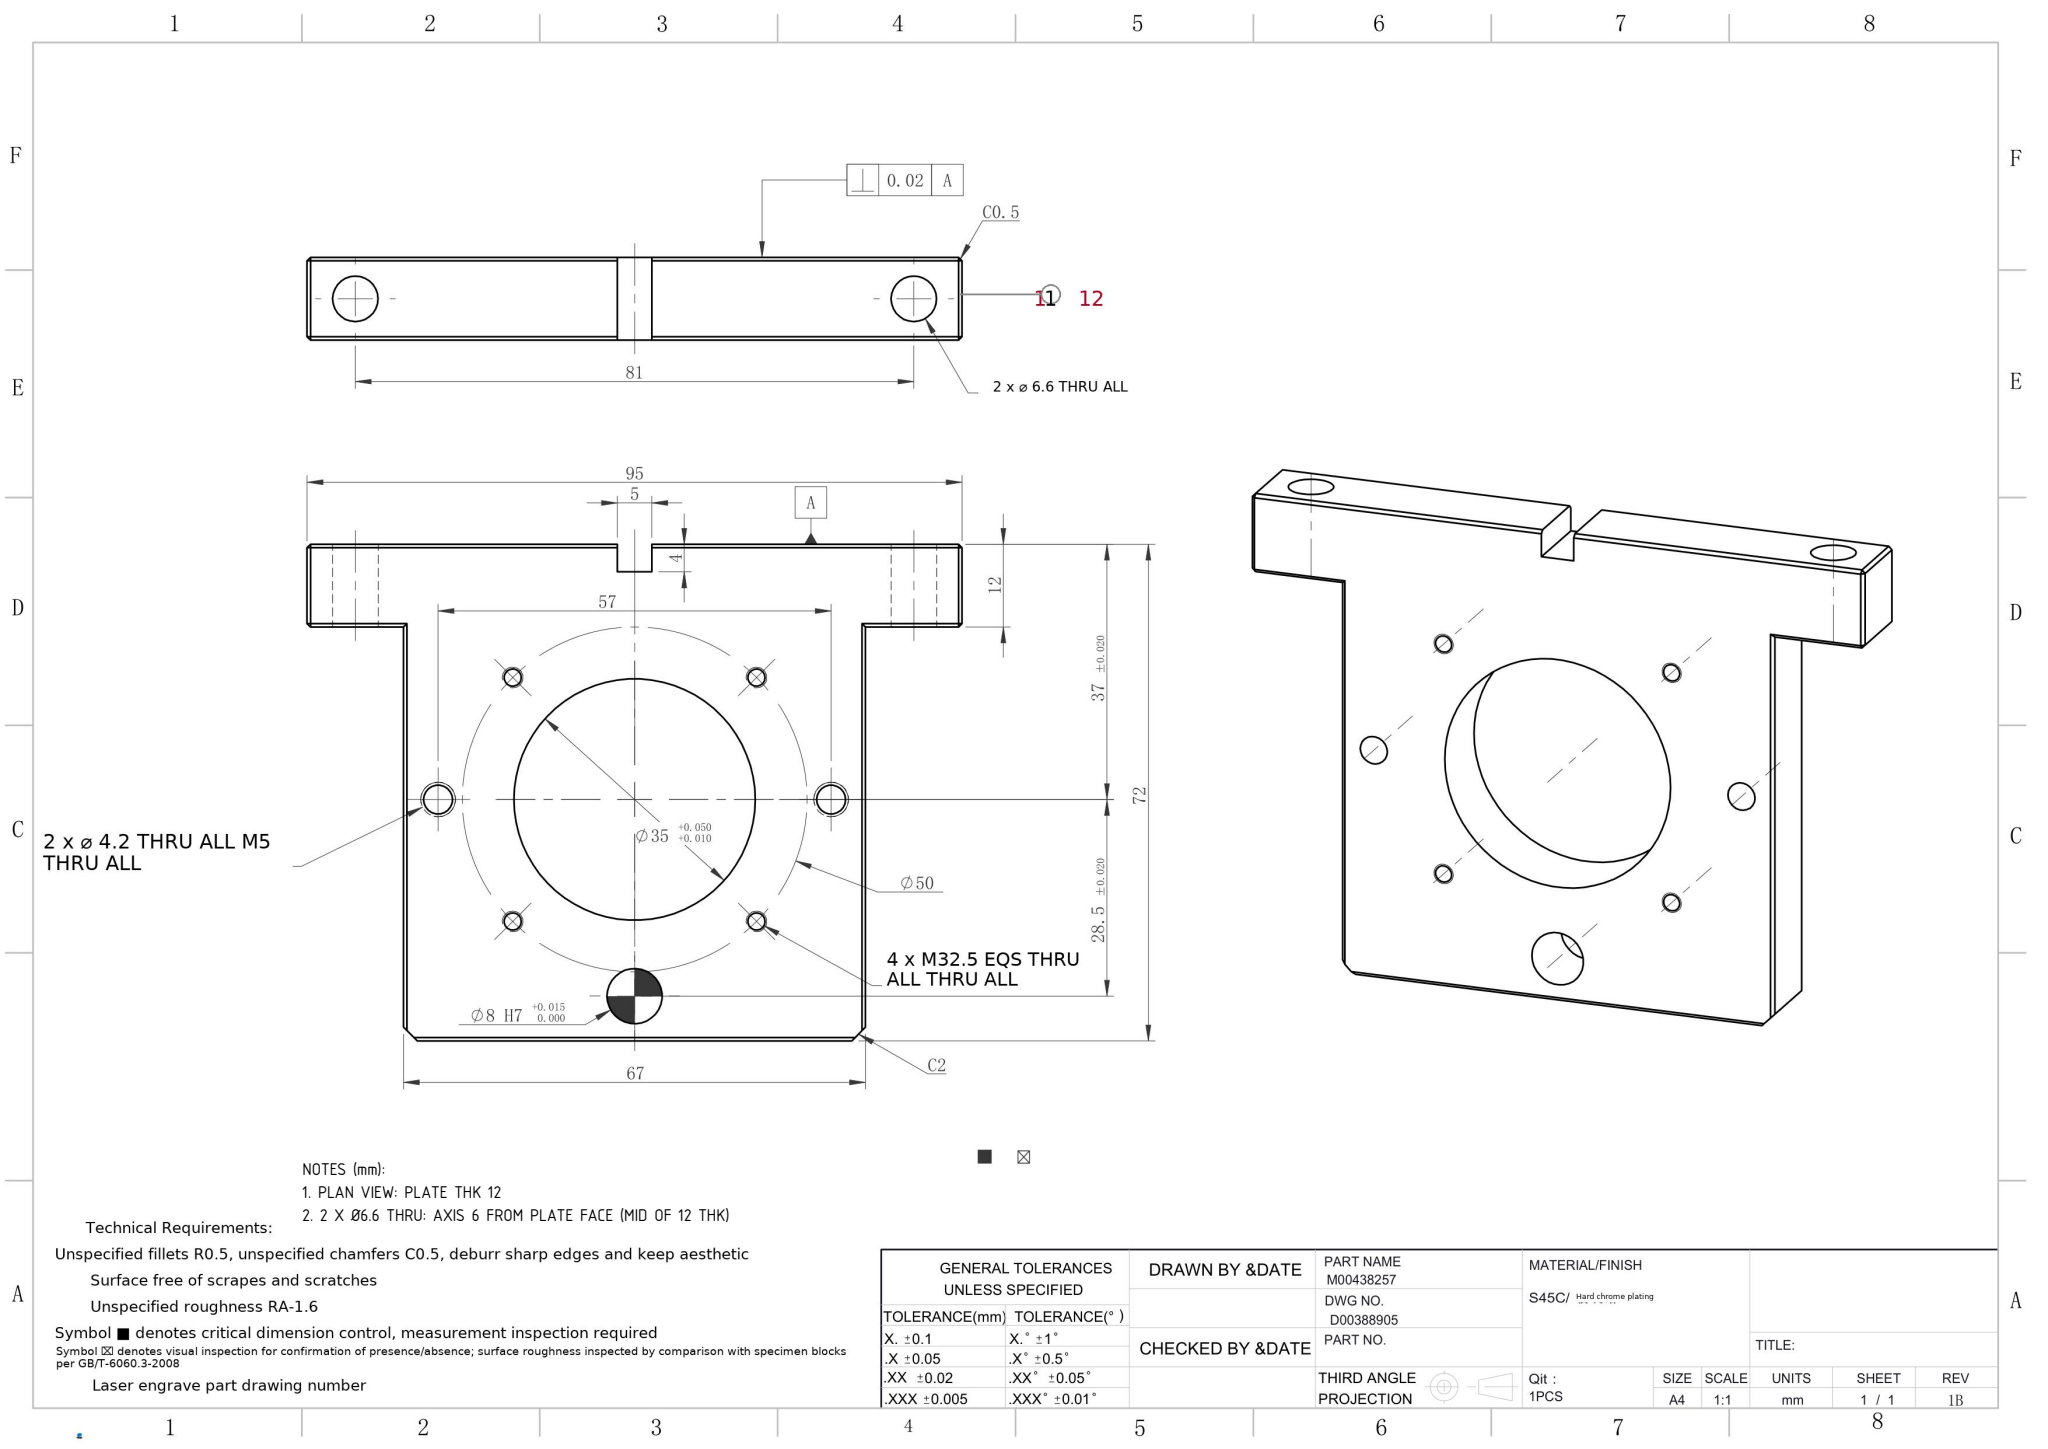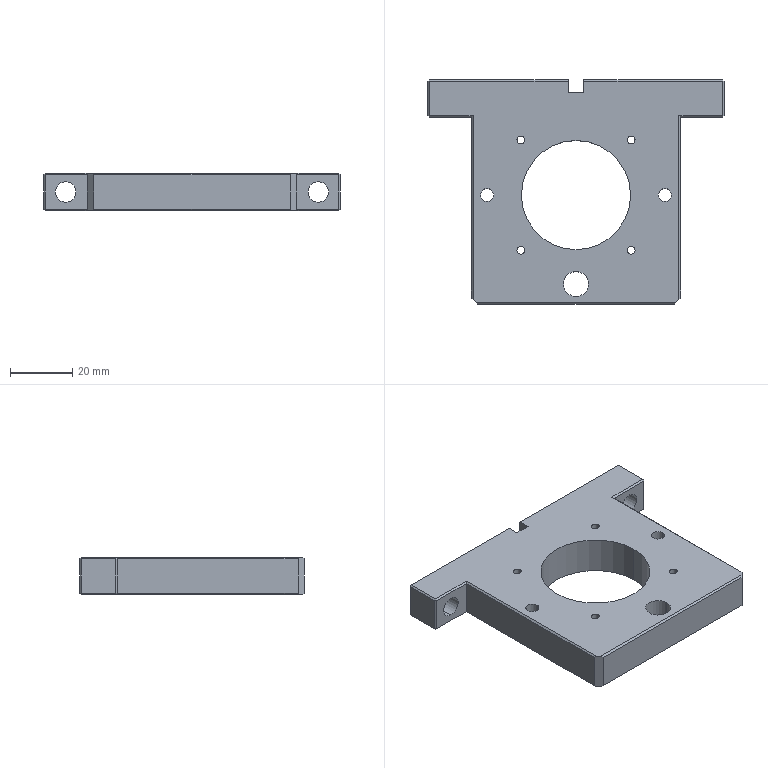Part | SolidWorks | mm | 1 solid | 70 faces | box 95 x 72 x 12 mm | volume 48006 mm3 | plane 46 | cylinder 20 | cone 4 | commonest cylinder face diameters 2.5 x8 4.2 x4 6.6 x4 8 x2 35 x2
Drawing notes:
PLAN VIEW: PLATE THK 12 | from the solid: bbox_xyz z = 12.0; planes z=0.0 and z=12.0
2 X Ø6.6 THRU: AXIS 6 FROM PLATE FACE (MID OF 12 THK) | from the solid: cylinders dia 6.6 axis y at z=6.0, thickness 12.0 (planes z=0/12)
build123d program:
from build123d import *

# Parameters (mm, degrees)
SKETCH1_W                   = 95
SKETCH1_H                   = 72
BOSS_EXTRUDE1_DEPTH         = 12
SKETCH2_R                   = 17.5
CUT_EXTRUDE1_DEPTH          = 61.797
M3_TAPPED_HOLE1_D           = 2.5
SKETCH9_W                   = 14
SKETCH9_H                   = 60
CUT_EXTRUDE2_DEPTH          = 61.797
M6_CLEARANCE_HOLE1_D        = 6.6
SKETCH14_W                  = 5
SKETCH14_H                  = 4
CUT_EXTRUDE3_DEPTH          = 61.797
CHAMFER2_SIZE               = 2
CHAMFER1_SIZE               = 0.5
M5_TAPPED_HOLE1_D           = 4.2
M5_TAPPED_HOLE1_CSINK_D     = 5.05
M5_TAPPED_HOLE1_CSINK_ANGLE = 90
SIZE_MM_DOWEL_PIN_HOLE1_D   = 8


with BuildPart() as part:
    # Sketch1 → Boss-Extrude1 (new body)
    with BuildSketch(Plane.XY):
        Rectangle(SKETCH1_W, SKETCH1_H)
    extrude(amount=BOSS_EXTRUDE1_DEPTH)

    # Sketch2 → Cut-Extrude1 (cut, through all)
    with BuildSketch(Plane.XY.offset(12)):
        with Locations((0, -1)):
            Circle(SKETCH2_R)
    extrude(amount=-CUT_EXTRUDE1_DEPTH, mode=Mode.SUBTRACT)

    # M3 Tapped Hole1 (through all)
    with Locations(Plane.XY.offset(12)):
        with Locations((-17.678, 16.678), (-17.678, -18.678), (17.678, 16.678), (17.678, -18.678)):
            Hole(M3_TAPPED_HOLE1_D / 2)

    # Sketch9 → Cut-Extrude2 (cut, through all)
    with BuildSketch(Plane.XY.offset(12)):
        with Locations((40.5, -6)):
            Rectangle(SKETCH9_W, SKETCH9_H)
        with Locations((-40.5, -6)):
            Rectangle(SKETCH9_W, SKETCH9_H)
    extrude(amount=-CUT_EXTRUDE2_DEPTH, mode=Mode.SUBTRACT)

    # M6 Clearance Hole1 (through all)
    with Locations(Plane(origin=(0, 24, 0), x_dir=(-1, 0, 0), z_dir=(0, -1, 0))):
        with Locations((40.5, -6), (-40.5, -6)):
            Hole(M6_CLEARANCE_HOLE1_D / 2)

    # Sketch14 → Cut-Extrude3 (cut, through all)
    with BuildSketch(Plane(origin=(0, 0, 0), x_dir=(-1, 0, 0), z_dir=(0, 0, -1))):
        with Locations((0, 34)):
            Rectangle(SKETCH14_W, SKETCH14_H)
    extrude(amount=-CUT_EXTRUDE3_DEPTH, mode=Mode.SUBTRACT)

    # Chamfer2
    chamfer2_edges = [part.edges().sort_by_distance(p)[0] for p in [
        (33.5, -36, 6),
        (-33.5, -36, 6),
    ]]
    chamfer(chamfer2_edges, length=CHAMFER2_SIZE)

    # Chamfer1
    chamfer1_edges = [part.edges().sort_by_distance(p)[0] for p in [
        (-47.5, 30, 12),
        (47.5, 30, 0),
        (47.5, 30, 12),
        (47.5, 24, 6),
        (-47.5, 30, 0),
        (33.5, -5, 0),
        (40.5, 24, 0),
        (40.5, 24, 12),
        (33.5, -5, 12),
        (25, 36, 0),
        (-40.5, 24, 0),
        (-47.5, 24, 6),
        (-40.5, 24, 12),
        (25, 36, 12),
        (-47.5, 36, 6),
        (47.5, 36, 6),
        (-25, 36, 0),
        (-25, 36, 12),
        (-33.5, -5, 12),
        (-33.5, -5, 0),
        (0, -36, 12),
        (0, -36, 0),
    ]]
    chamfer(chamfer1_edges, length=CHAMFER1_SIZE)

    # M5 Tapped Hole1 (through all)
    with Locations(Plane(origin=(0, 0, 0), x_dir=(-1, 0, 0), z_dir=(0, 0, -1))):
        with Locations((28.5, -1), (-28.5, -1)):
            CounterSinkHole(M5_TAPPED_HOLE1_D / 2, M5_TAPPED_HOLE1_CSINK_D / 2, counter_sink_angle=M5_TAPPED_HOLE1_CSINK_ANGLE)

    # Size mm Dowel Pin Hole1 (through all)
    with Locations(Plane(origin=(0, 0, 0), x_dir=(-1, 0, 0), z_dir=(0, 0, -1))):
        with Locations((0, -29.5)):
            Hole(SIZE_MM_DOWEL_PIN_HOLE1_D / 2)


solid = part.part